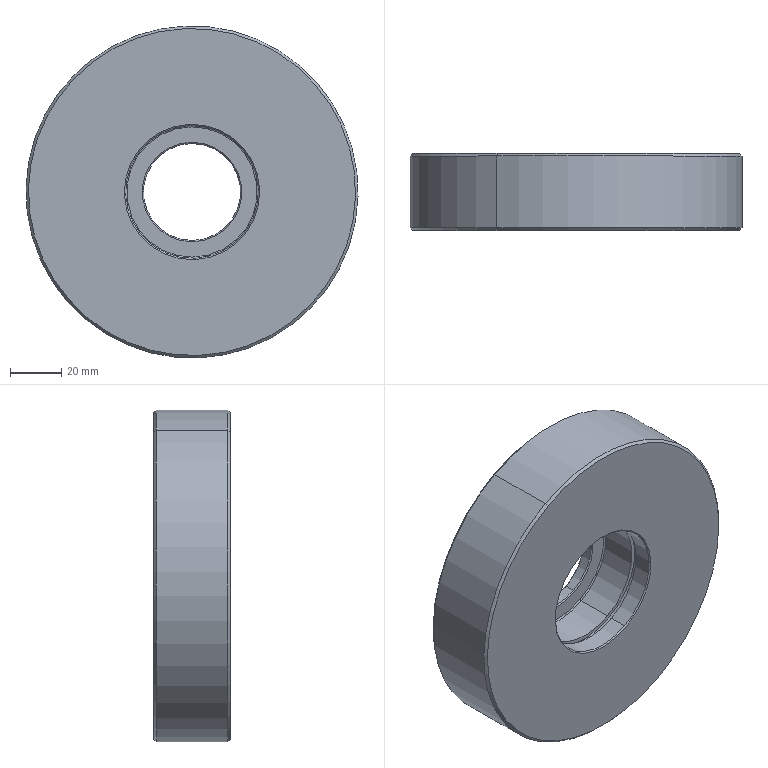Component | SolidWorks | Yk1.5.4NylonRoller-1 | 1 solid | 27 faces | box 130 x 30 x 130 mm | volume 338430 mm3 | cylinder 10 | cone 10 | plane 5 | torus 2 | commonest cylinder face diameters 52 x4 55 x2 130 x2 38 x2 | material MC Nylon
build123d program:
from build123d import *

# Parameters (mm, degrees)
SKETCH1_R           = 65
SKETCH1_R_2         = 19
BOSS_EXTRUDE1_DEPTH = 30
CHAMFER1_SIZE       = 1
SKETCH2_R           = 26
CUT_EXTRUDE2_DEPTH  = 25
CHAMFER2_SIZE       = 0.5
SKETCH3_W           = 27.5
SKETCH3_H           = 2.2
FILLET1_R           = 0.5


with BuildPart() as part:
    # Sketch1 → Boss-Extrude1 (new body)
    with BuildSketch(Plane(origin=(0, 0, 0), x_dir=(1, 0, 0), z_dir=(0, 1, 0))):
        with Locations(Location((0, 0, 0), (0, 0, 270))):
            Circle(SKETCH1_R)
        with Locations(Location((0, 0, 0), (0, 0, 270))):
            Circle(SKETCH1_R_2, mode=Mode.SUBTRACT)
    extrude(amount=BOSS_EXTRUDE1_DEPTH)

    # Chamfer1
    chamfer1_edges = [part.edges().sort_by_distance(p)[0] for p in [
        (0, 0, -65),
        (0, 30, -65),
    ]]
    chamfer(chamfer1_edges, length=CHAMFER1_SIZE)

    # Sketch2 → Cut-Extrude2 (cut)
    with BuildSketch(Plane(origin=(0, 30, 0), x_dir=(1, 0, 0), z_dir=(0, 1, 0))):
        with Locations(Location((0, 0, 0), (0, 0, 270))):
            Circle(SKETCH2_R)
    extrude(amount=-CUT_EXTRUDE2_DEPTH, mode=Mode.SUBTRACT)

    # Chamfer2
    chamfer2_edges = [part.edges().sort_by_distance(p)[0] for p in [
        (0, 5, -19),
        (0, 30, -26),
        (0, 0, -19),
    ]]
    chamfer(chamfer2_edges, length=CHAMFER2_SIZE)

    # Sketch3 → Cut-Revolve1 (revolve, cut)
    with BuildSketch(Plane.XY, mode=Mode.PRIVATE) as cut_revolve1_sk:
        with Locations((13.75, 21.1)):
            Rectangle(SKETCH3_W, SKETCH3_H)
    revolve(cut_revolve1_sk.sketch.rotate(Axis((0, 0, 0), (0, 1, 0)), 270), axis=Axis((0, 0, 0), (0, 1, 0)), mode=Mode.SUBTRACT)

    # Fillet1
    fillet1_edges = [part.edges().sort_by_distance(p)[0] for p in [
        (0, 5, -26),
    ]]
    fillet(fillet1_edges, radius=FILLET1_R)


solid = part.part

# Placed as in the assembly
solid = solid.moved(Location((98.534, -20, 23.559), (180, 0, 0)))
STEP:
#1=CARTESIAN_POINT('',(4.358,-0.9843,0.04503));
#2=VERTEX_POINT('',#1);
#3=CARTESIAN_POINT('',(3.401,-0.9843,1.81));
#4=VERTEX_POINT('',#3);
#5=CARTESIAN_POINT('',(3.879,-0.9843,0.9275));
#6=DIRECTION('',(0.,-1.,-0.));
#7=DIRECTION('',(-0.4768,0.,0.879));
#8=AXIS2_PLACEMENT_3D('',#5,#6,#7);
#9=CIRCLE('',#8,1.004);
#10=EDGE_CURVE('',#2,#4,#9,.T.);
#11=ORIENTED_EDGE('',*,*,#10,.F.);
#12=CARTESIAN_POINT('',(4.367,-1.004,0.02773));
#13=VERTEX_POINT('',#12);
#14=CARTESIAN_POINT('',(4.358,-1.004,0.04503));
#15=DIRECTION('',(-0.879,-0.,-0.4768));
#16=DIRECTION('',(-0.4768,0.,0.879));
#17=AXIS2_PLACEMENT_3D('',#14,#15,#16);
#18=CIRCLE('',#17,0.01969);
#19=EDGE_CURVE('',#2,#13,#18,.T.);
#20=ORIENTED_EDGE('',*,*,#19,.T.);
#21=CARTESIAN_POINT('',(3.391,-1.004,1.827));
#22=VERTEX_POINT('',#21);
#23=CARTESIAN_POINT('',(3.879,-1.004,0.9275));
#24=DIRECTION('',(-0.,1.,0.));
#25=DIRECTION('',(-0.4768,0.,0.879));
#26=AXIS2_PLACEMENT_3D('',#23,#24,#25);
#27=CIRCLE('',#26,1.024);
#28=EDGE_CURVE('',#22,#13,#27,.T.);
#29=ORIENTED_EDGE('',*,*,#28,.F.);
#30=CARTESIAN_POINT('',(3.401,-1.004,1.81));
#31=DIRECTION('',(0.879,0.,0.4768));
#32=DIRECTION('',(0.4768,0.,-0.879));
#33=AXIS2_PLACEMENT_3D('',#30,#31,#32);
#34=CIRCLE('',#33,0.01969);
#35=EDGE_CURVE('',#4,#22,#34,.T.);
#36=ORIENTED_EDGE('',*,*,#35,.F.);
#37=EDGE_LOOP('',(#11,#20,#29,#36));
#38=FACE_OUTER_BOUND('',#37,.T.);
#39=CARTESIAN_POINT('',(3.879,-1.004,0.9275));
#40=DIRECTION('',(0.,-1.,-0.));
#41=DIRECTION('',(-0.4768,-0.,0.879));
#42=AXIS2_PLACEMENT_3D('',#39,#40,#41);
#43=TOROIDAL_SURFACE('',#42,1.004,0.01969);
#44=ADVANCED_FACE('',(#38),#43,.F.);
#45=CARTESIAN_POINT('',(3.363,-1.661,1.879));
#46=VERTEX_POINT('',#45);
#47=CARTESIAN_POINT('',(4.395,-1.661,-0.02418));
#48=VERTEX_POINT('',#47);
#49=CARTESIAN_POINT('',(3.879,-1.661,0.9275));
#50=DIRECTION('',(-0.,1.,0.));
#51=DIRECTION('',(0.4768,0.,-0.879));
#52=AXIS2_PLACEMENT_3D('',#49,#50,#51);
#53=CIRCLE('',#52,1.083);
#54=EDGE_CURVE('',#46,#48,#53,.T.);
#55=ORIENTED_EDGE('',*,*,#54,.F.);
#56=CARTESIAN_POINT('',(3.363,-1.575,1.879));
#57=VERTEX_POINT('',#56);
#58=CARTESIAN_POINT('',(3.363,-0.7874,1.879));
#59=DIRECTION('',(-0.,1.,0.));
#60=VECTOR('',#59,39.37);
#61=LINE('',#58,#60);
#62=EDGE_CURVE('',#46,#57,#61,.T.);
#63=ORIENTED_EDGE('',*,*,#62,.T.);
#64=CARTESIAN_POINT('',(4.395,-1.575,-0.02418));
#65=VERTEX_POINT('',#64);
#66=CARTESIAN_POINT('',(3.879,-1.575,0.9275));
#67=DIRECTION('',(-0.,1.,0.));
#68=DIRECTION('',(0.4768,0.,-0.879));
#69=AXIS2_PLACEMENT_3D('',#66,#67,#68);
#70=CIRCLE('',#69,1.083);
#71=EDGE_CURVE('',#57,#65,#70,.T.);
#72=ORIENTED_EDGE('',*,*,#71,.T.);
#73=CARTESIAN_POINT('',(4.395,-0.7874,-0.02418));
#74=DIRECTION('',(-0.,1.,0.));
#75=VECTOR('',#74,39.37);
#76=LINE('',#73,#75);
#77=EDGE_CURVE('',#48,#65,#76,.T.);
#78=ORIENTED_EDGE('',*,*,#77,.F.);
#79=EDGE_LOOP('',(#55,#63,#72,#78));
#80=FACE_OUTER_BOUND('',#79,.T.);
#81=CARTESIAN_POINT('',(3.879,-0.7874,0.9275));
#82=DIRECTION('',(-0.,1.,0.));
#83=DIRECTION('',(0.4768,0.,-0.879));
#84=AXIS2_PLACEMENT_3D('',#81,#82,#83);
#85=CYLINDRICAL_SURFACE('',#84,1.083);
#86=ADVANCED_FACE('',(#80),#85,.F.);
#87=CARTESIAN_POINT('',(3.523,-0.8071,1.585));
#88=VERTEX_POINT('',#87);
#89=CARTESIAN_POINT('',(4.236,-0.8071,0.27));
#90=VERTEX_POINT('',#89);
#91=CARTESIAN_POINT('',(3.879,-0.8071,0.9275));
#92=DIRECTION('',(-0.,1.,0.));
#93=DIRECTION('',(-0.4768,0.,0.879));
#94=AXIS2_PLACEMENT_3D('',#91,#92,#93);
#95=CIRCLE('',#94,0.748);
#96=EDGE_CURVE('',#88,#90,#95,.T.);
#97=ORIENTED_EDGE('',*,*,#96,.F.);
#98=CARTESIAN_POINT('',(3.513,-0.7874,1.602));
#99=VERTEX_POINT('',#98);
#100=CARTESIAN_POINT('',(3.513,-0.7874,1.602));
#101=DIRECTION('',(-0.3371,0.7071,0.6216));
#102=VECTOR('',#101,39.37);
#103=LINE('',#100,#102);
#104=EDGE_CURVE('',#88,#99,#103,.T.);
#105=ORIENTED_EDGE('',*,*,#104,.T.);
#106=CARTESIAN_POINT('',(4.245,-0.7874,0.2527));
#107=VERTEX_POINT('',#106);
#108=CARTESIAN_POINT('',(3.879,-0.7874,0.9275));
#109=DIRECTION('',(0.,-1.,-0.));
#110=DIRECTION('',(-0.4768,0.,0.879));
#111=AXIS2_PLACEMENT_3D('',#108,#109,#110);
#112=CIRCLE('',#111,0.7677);
#113=EDGE_CURVE('',#107,#99,#112,.T.);
#114=ORIENTED_EDGE('',*,*,#113,.F.);
#115=CARTESIAN_POINT('',(4.245,-0.7874,0.2527));
#116=DIRECTION('',(0.3371,0.7071,-0.6216));
#117=VECTOR('',#116,39.37);
#118=LINE('',#115,#117);
#119=EDGE_CURVE('',#90,#107,#118,.T.);
#120=ORIENTED_EDGE('',*,*,#119,.F.);
#121=EDGE_LOOP('',(#97,#105,#114,#120));
#122=FACE_OUTER_BOUND('',#121,.T.);
#123=CARTESIAN_POINT('',(3.879,-0.7874,0.9275));
#124=DIRECTION('',(-0.,1.,0.));
#125=DIRECTION('',(0.4768,0.,-0.879));
#126=AXIS2_PLACEMENT_3D('',#123,#124,#125);
#127=CONICAL_SURFACE('',#126,0.7677,0.7854);
#128=ADVANCED_FACE('',(#122),#127,.F.);
#129=CARTESIAN_POINT('',(4.236,-0.9646,0.27));
#130=VERTEX_POINT('',#129);
#131=CARTESIAN_POINT('',(3.523,-0.9646,1.585));
#132=VERTEX_POINT('',#131);
#133=CARTESIAN_POINT('',(3.879,-0.9646,0.9275));
#134=DIRECTION('',(0.,-1.,-0.));
#135=DIRECTION('',(-0.4768,0.,0.879));
#136=AXIS2_PLACEMENT_3D('',#133,#134,#135);
#137=CIRCLE('',#136,0.748);
#138=EDGE_CURVE('',#130,#132,#137,.T.);
#139=ORIENTED_EDGE('',*,*,#138,.F.);
#140=CARTESIAN_POINT('',(4.245,-0.9843,0.2527));
#141=VERTEX_POINT('',#140);
#142=CARTESIAN_POINT('',(4.236,-0.9646,0.27));
#143=DIRECTION('',(0.3371,-0.7071,-0.6216));
#144=VECTOR('',#143,39.37);
#145=LINE('',#142,#144);
#146=EDGE_CURVE('',#130,#141,#145,.T.);
#147=ORIENTED_EDGE('',*,*,#146,.T.);
#148=CARTESIAN_POINT('',(3.513,-0.9843,1.602));
#149=VERTEX_POINT('',#148);
#150=CARTESIAN_POINT('',(3.879,-0.9843,0.9275));
#151=DIRECTION('',(-0.,1.,0.));
#152=DIRECTION('',(-0.4768,0.,0.879));
#153=AXIS2_PLACEMENT_3D('',#150,#151,#152);
#154=CIRCLE('',#153,0.7677);
#155=EDGE_CURVE('',#149,#141,#154,.T.);
#156=ORIENTED_EDGE('',*,*,#155,.F.);
#157=CARTESIAN_POINT('',(3.523,-0.9646,1.585));
#158=DIRECTION('',(-0.3371,-0.7071,0.6216));
#159=VECTOR('',#158,39.37);
#160=LINE('',#157,#159);
#161=EDGE_CURVE('',#132,#149,#160,.T.);
#162=ORIENTED_EDGE('',*,*,#161,.F.);
#163=EDGE_LOOP('',(#139,#147,#156,#162));
#164=FACE_OUTER_BOUND('',#163,.T.);
#165=CARTESIAN_POINT('',(3.879,-0.9646,0.9275));
#166=DIRECTION('',(0.,-1.,-0.));
#167=DIRECTION('',(-0.4768,0.,0.879));
#168=AXIS2_PLACEMENT_3D('',#165,#166,#167);
#169=CONICAL_SURFACE('',#168,0.748,0.7854);
#170=ADVANCED_FACE('',(#164),#169,.F.);
#171=CARTESIAN_POINT('',(4.367,-1.949,0.02773));
#172=VERTEX_POINT('',#171);
#173=CARTESIAN_POINT('',(3.391,-1.949,1.827));
#174=VERTEX_POINT('',#173);
#175=CARTESIAN_POINT('',(3.879,-1.949,0.9275));
#176=DIRECTION('',(0.,-1.,-0.));
#177=DIRECTION('',(-0.4768,0.,0.879));
#178=AXIS2_PLACEMENT_3D('',#175,#176,#177);
#179=CIRCLE('',#178,1.024);
#180=EDGE_CURVE('',#172,#174,#179,.T.);
#181=ORIENTED_EDGE('',*,*,#180,.F.);
#182=CARTESIAN_POINT('',(4.377,-1.969,0.01042));
#183=VERTEX_POINT('',#182);
#184=CARTESIAN_POINT('',(4.367,-1.949,0.02773));
#185=DIRECTION('',(0.3371,-0.7071,-0.6216));
#186=VECTOR('',#185,39.37);
#187=LINE('',#184,#186);
#188=EDGE_CURVE('',#172,#183,#187,.T.);
#189=ORIENTED_EDGE('',*,*,#188,.T.);
#190=CARTESIAN_POINT('',(3.382,-1.969,1.845));
#191=VERTEX_POINT('',#190);
#192=CARTESIAN_POINT('',(3.879,-1.969,0.9275));
#193=DIRECTION('',(-0.,1.,0.));
#194=DIRECTION('',(-0.4768,0.,0.879));
#195=AXIS2_PLACEMENT_3D('',#192,#193,#194);
#196=CIRCLE('',#195,1.043);
#197=EDGE_CURVE('',#191,#183,#196,.T.);
#198=ORIENTED_EDGE('',*,*,#197,.F.);
#199=CARTESIAN_POINT('',(3.391,-1.949,1.827));
#200=DIRECTION('',(-0.3371,-0.7071,0.6216));
#201=VECTOR('',#200,39.37);
#202=LINE('',#199,#201);
#203=EDGE_CURVE('',#174,#191,#202,.T.);
#204=ORIENTED_EDGE('',*,*,#203,.F.);
#205=EDGE_LOOP('',(#181,#189,#198,#204));
#206=FACE_OUTER_BOUND('',#205,.T.);
#207=CARTESIAN_POINT('',(3.879,-1.949,0.9275));
#208=DIRECTION('',(0.,-1.,-0.));
#209=DIRECTION('',(-0.4768,0.,0.879));
#210=AXIS2_PLACEMENT_3D('',#207,#208,#209);
#211=CONICAL_SURFACE('',#210,1.024,0.7854);
#212=ADVANCED_FACE('',(#206),#211,.F.);
#213=CARTESIAN_POINT('',(3.391,-1.661,1.827));
#214=VERTEX_POINT('',#213);
#215=CARTESIAN_POINT('',(4.367,-1.661,0.02773));
#216=VERTEX_POINT('',#215);
#217=CARTESIAN_POINT('',(3.879,-1.661,0.9275));
#218=DIRECTION('',(-0.,1.,0.));
#219=DIRECTION('',(-0.4768,0.,0.879));
#220=AXIS2_PLACEMENT_3D('',#217,#218,#219);
#221=CIRCLE('',#220,1.024);
#222=EDGE_CURVE('',#214,#216,#221,.T.);
#223=ORIENTED_EDGE('',*,*,#222,.T.);
#224=CARTESIAN_POINT('',(4.367,-0.9843,0.02773));
#225=DIRECTION('',(0.,-1.,-0.));
#226=VECTOR('',#225,39.37);
#227=LINE('',#224,#226);
#228=EDGE_CURVE('',#216,#172,#227,.T.);
#229=ORIENTED_EDGE('',*,*,#228,.T.);
#230=ORIENTED_EDGE('',*,*,#180,.T.);
#231=CARTESIAN_POINT('',(3.391,-0.9843,1.827));
#232=DIRECTION('',(0.,-1.,-0.));
#233=VECTOR('',#232,39.37);
#234=LINE('',#231,#233);
#235=EDGE_CURVE('',#214,#174,#234,.T.);
#236=ORIENTED_EDGE('',*,*,#235,.F.);
#237=EDGE_LOOP('',(#223,#229,#230,#236));
#238=FACE_OUTER_BOUND('',#237,.T.);
#239=CARTESIAN_POINT('',(3.879,-0.9843,0.9275));
#240=DIRECTION('',(0.,-1.,-0.));
#241=DIRECTION('',(-0.4768,0.,0.879));
#242=AXIS2_PLACEMENT_3D('',#239,#240,#241);
#243=CYLINDRICAL_SURFACE('',#242,1.024);
#244=ADVANCED_FACE('',(#238),#243,.F.);
#245=CARTESIAN_POINT('',(2.678,-1.969,3.142));
#246=VERTEX_POINT('',#245);
#247=CARTESIAN_POINT('',(5.081,-1.969,-1.287));
#248=VERTEX_POINT('',#247);
#249=CARTESIAN_POINT('',(3.879,-1.969,0.9275));
#250=DIRECTION('',(0.,-1.,-0.));
#251=DIRECTION('',(-0.4768,0.,0.879));
#252=AXIS2_PLACEMENT_3D('',#249,#250,#251);
#253=CIRCLE('',#252,2.52);
#254=EDGE_CURVE('',#246,#248,#253,.T.);
#255=ORIENTED_EDGE('',*,*,#254,.F.);
#256=CARTESIAN_POINT('',(2.659,-1.929,3.177));
#257=VERTEX_POINT('',#256);
#258=CARTESIAN_POINT('',(2.678,-1.969,3.142));
#259=DIRECTION('',(-0.3371,0.7071,0.6216));
#260=VECTOR('',#259,39.37);
#261=LINE('',#258,#260);
#262=EDGE_CURVE('',#246,#257,#261,.T.);
#263=ORIENTED_EDGE('',*,*,#262,.T.);
#264=CARTESIAN_POINT('',(5.099,-1.929,-1.322));
#265=VERTEX_POINT('',#264);
#266=CARTESIAN_POINT('',(3.879,-1.929,0.9275));
#267=DIRECTION('',(-0.,1.,0.));
#268=DIRECTION('',(-0.4768,0.,0.879));
#269=AXIS2_PLACEMENT_3D('',#266,#267,#268);
#270=CIRCLE('',#269,2.559);
#271=EDGE_CURVE('',#265,#257,#270,.T.);
#272=ORIENTED_EDGE('',*,*,#271,.F.);
#273=CARTESIAN_POINT('',(5.081,-1.969,-1.287));
#274=DIRECTION('',(0.3371,0.7071,-0.6216));
#275=VECTOR('',#274,39.37);
#276=LINE('',#273,#275);
#277=EDGE_CURVE('',#248,#265,#276,.T.);
#278=ORIENTED_EDGE('',*,*,#277,.F.);
#279=EDGE_LOOP('',(#255,#263,#272,#278));
#280=FACE_OUTER_BOUND('',#279,.T.);
#281=CARTESIAN_POINT('',(3.879,-1.969,0.9275));
#282=DIRECTION('',(-0.,1.,0.));
#283=DIRECTION('',(0.4768,0.,-0.879));
#284=AXIS2_PLACEMENT_3D('',#281,#282,#283);
#285=CONICAL_SURFACE('',#284,2.52,0.7854);
#286=ADVANCED_FACE('',(#280),#285,.T.);
#287=CARTESIAN_POINT('',(5.081,-0.7874,-1.287));
#288=VERTEX_POINT('',#287);
#289=CARTESIAN_POINT('',(2.678,-0.7874,3.142));
#290=VERTEX_POINT('',#289);
#291=CARTESIAN_POINT('',(3.879,-0.7874,0.9275));
#292=DIRECTION('',(-0.,1.,0.));
#293=DIRECTION('',(-0.4768,0.,0.879));
#294=AXIS2_PLACEMENT_3D('',#291,#292,#293);
#295=CIRCLE('',#294,2.52);
#296=EDGE_CURVE('',#288,#290,#295,.T.);
#297=ORIENTED_EDGE('',*,*,#296,.F.);
#298=CARTESIAN_POINT('',(5.099,-0.8268,-1.322));
#299=VERTEX_POINT('',#298);
#300=CARTESIAN_POINT('',(5.099,-0.8268,-1.322));
#301=DIRECTION('',(0.3371,-0.7071,-0.6216));
#302=VECTOR('',#301,39.37);
#303=LINE('',#300,#302);
#304=EDGE_CURVE('',#288,#299,#303,.T.);
#305=ORIENTED_EDGE('',*,*,#304,.T.);
#306=CARTESIAN_POINT('',(2.659,-0.8268,3.177));
#307=VERTEX_POINT('',#306);
#308=CARTESIAN_POINT('',(3.879,-0.8268,0.9275));
#309=DIRECTION('',(0.,-1.,-0.));
#310=DIRECTION('',(-0.4768,0.,0.879));
#311=AXIS2_PLACEMENT_3D('',#308,#309,#310);
#312=CIRCLE('',#311,2.559);
#313=EDGE_CURVE('',#307,#299,#312,.T.);
#314=ORIENTED_EDGE('',*,*,#313,.F.);
#315=CARTESIAN_POINT('',(2.659,-0.8268,3.177));
#316=DIRECTION('',(-0.3371,-0.7071,0.6216));
#317=VECTOR('',#316,39.37);
#318=LINE('',#315,#317);
#319=EDGE_CURVE('',#290,#307,#318,.T.);
#320=ORIENTED_EDGE('',*,*,#319,.F.);
#321=EDGE_LOOP('',(#297,#305,#314,#320));
#322=FACE_OUTER_BOUND('',#321,.T.);
#323=CARTESIAN_POINT('',(3.879,-0.8268,0.9275));
#324=DIRECTION('',(0.,-1.,-0.));
#325=DIRECTION('',(-0.4768,0.,0.879));
#326=AXIS2_PLACEMENT_3D('',#323,#324,#325);
#327=CONICAL_SURFACE('',#326,2.559,0.7854);
#328=ADVANCED_FACE('',(#322),#327,.T.);
#329=ORIENTED_EDGE('',*,*,#271,.T.);
#330=CARTESIAN_POINT('',(2.659,-1.969,3.177));
#331=DIRECTION('',(-0.,1.,0.));
#332=VECTOR('',#331,39.37);
#333=LINE('',#330,#332);
#334=EDGE_CURVE('',#257,#307,#333,.T.);
#335=ORIENTED_EDGE('',*,*,#334,.T.);
#336=ORIENTED_EDGE('',*,*,#313,.T.);
#337=CARTESIAN_POINT('',(5.099,-1.969,-1.322));
#338=DIRECTION('',(-0.,1.,0.));
#339=VECTOR('',#338,39.37);
#340=LINE('',#337,#339);
#341=EDGE_CURVE('',#265,#299,#340,.T.);
#342=ORIENTED_EDGE('',*,*,#341,.F.);
#343=EDGE_LOOP('',(#329,#335,#336,#342));
#344=FACE_OUTER_BOUND('',#343,.T.);
#345=CARTESIAN_POINT('',(3.879,-1.969,0.9275));
#346=DIRECTION('',(-0.,1.,0.));
#347=DIRECTION('',(0.4768,0.,-0.879));
#348=AXIS2_PLACEMENT_3D('',#345,#346,#347);
#349=CYLINDRICAL_SURFACE('',#348,2.559);
#350=ADVANCED_FACE('',(#344),#349,.T.);
#351=ORIENTED_EDGE('',*,*,#138,.T.);
#352=CARTESIAN_POINT('',(3.523,-1.969,1.585));
#353=DIRECTION('',(-0.,1.,0.));
#354=VECTOR('',#353,39.37);
#355=LINE('',#352,#354);
#356=EDGE_CURVE('',#132,#88,#355,.T.);
#357=ORIENTED_EDGE('',*,*,#356,.T.);
#358=ORIENTED_EDGE('',*,*,#96,.T.);
#359=CARTESIAN_POINT('',(4.236,-1.969,0.27));
#360=DIRECTION('',(-0.,1.,0.));
#361=VECTOR('',#360,39.37);
#362=LINE('',#359,#361);
#363=EDGE_CURVE('',#130,#90,#362,.T.);
#364=ORIENTED_EDGE('',*,*,#363,.F.);
#365=EDGE_LOOP('',(#351,#357,#358,#364));
#366=FACE_OUTER_BOUND('',#365,.T.);
#367=CARTESIAN_POINT('',(3.879,-1.969,0.9275));
#368=DIRECTION('',(-0.,1.,0.));
#369=DIRECTION('',(0.4768,0.,-0.879));
#370=AXIS2_PLACEMENT_3D('',#367,#368,#369);
#371=CYLINDRICAL_SURFACE('',#370,0.748);
#372=ADVANCED_FACE('',(#366),#371,.F.);
#373=ORIENTED_EDGE('',*,*,#28,.T.);
#374=CARTESIAN_POINT('',(4.367,-1.575,0.02773));
#375=VERTEX_POINT('',#374);
#376=CARTESIAN_POINT('',(4.367,-0.9843,0.02773));
#377=DIRECTION('',(0.,-1.,-0.));
#378=VECTOR('',#377,39.37);
#379=LINE('',#376,#378);
#380=EDGE_CURVE('',#13,#375,#379,.T.);
#381=ORIENTED_EDGE('',*,*,#380,.T.);
#382=CARTESIAN_POINT('',(3.391,-1.575,1.827));
#383=VERTEX_POINT('',#382);
#384=CARTESIAN_POINT('',(3.879,-1.575,0.9275));
#385=DIRECTION('',(0.,-1.,-0.));
#386=DIRECTION('',(0.4768,0.,-0.879));
#387=AXIS2_PLACEMENT_3D('',#384,#385,#386);
#388=CIRCLE('',#387,1.024);
#389=EDGE_CURVE('',#375,#383,#388,.T.);
#390=ORIENTED_EDGE('',*,*,#389,.T.);
#391=CARTESIAN_POINT('',(3.391,-0.9843,1.827));
#392=DIRECTION('',(0.,-1.,-0.));
#393=VECTOR('',#392,39.37);
#394=LINE('',#391,#393);
#395=EDGE_CURVE('',#22,#383,#394,.T.);
#396=ORIENTED_EDGE('',*,*,#395,.F.);
#397=EDGE_LOOP('',(#373,#381,#390,#396));
#398=FACE_OUTER_BOUND('',#397,.T.);
#399=CARTESIAN_POINT('',(3.879,-0.9843,0.9275));
#400=DIRECTION('',(0.,-1.,-0.));
#401=DIRECTION('',(-0.4768,0.,0.879));
#402=AXIS2_PLACEMENT_3D('',#399,#400,#401);
#403=CYLINDRICAL_SURFACE('',#402,1.024);
#404=ADVANCED_FACE('',(#398),#403,.F.);
#405=ORIENTED_EDGE('',*,*,#380,.F.);
#406=CARTESIAN_POINT('',(3.879,-1.004,0.9275));
#407=DIRECTION('',(-0.,1.,0.));
#408=DIRECTION('',(-0.4768,0.,0.879));
#409=AXIS2_PLACEMENT_3D('',#406,#407,#408);
#410=CIRCLE('',#409,1.024);
#411=EDGE_CURVE('',#13,#22,#410,.T.);
#412=ORIENTED_EDGE('',*,*,#411,.T.);
#413=ORIENTED_EDGE('',*,*,#395,.T.);
#414=CARTESIAN_POINT('',(3.879,-1.575,0.9275));
#415=DIRECTION('',(0.,-1.,-0.));
#416=DIRECTION('',(0.4768,0.,-0.879));
#417=AXIS2_PLACEMENT_3D('',#414,#415,#416);
#418=CIRCLE('',#417,1.024);
#419=EDGE_CURVE('',#383,#375,#418,.T.);
#420=ORIENTED_EDGE('',*,*,#419,.T.);
#421=EDGE_LOOP('',(#405,#412,#413,#420));
#422=FACE_OUTER_BOUND('',#421,.T.);
#423=CARTESIAN_POINT('',(3.879,-0.9843,0.9275));
#424=DIRECTION('',(0.,-1.,-0.));
#425=DIRECTION('',(-0.4768,0.,0.879));
#426=AXIS2_PLACEMENT_3D('',#423,#424,#425);
#427=CYLINDRICAL_SURFACE('',#426,1.024);
#428=ADVANCED_FACE('',(#422),#427,.F.);
#429=ORIENTED_EDGE('',*,*,#356,.F.);
#430=CARTESIAN_POINT('',(3.879,-0.9646,0.9275));
#431=DIRECTION('',(0.,-1.,-0.));
#432=DIRECTION('',(-0.4768,0.,0.879));
#433=AXIS2_PLACEMENT_3D('',#430,#431,#432);
#434=CIRCLE('',#433,0.748);
#435=EDGE_CURVE('',#132,#130,#434,.T.);
#436=ORIENTED_EDGE('',*,*,#435,.T.);
#437=ORIENTED_EDGE('',*,*,#363,.T.);
#438=CARTESIAN_POINT('',(3.879,-0.8071,0.9275));
#439=DIRECTION('',(-0.,1.,0.));
#440=DIRECTION('',(-0.4768,0.,0.879));
#441=AXIS2_PLACEMENT_3D('',#438,#439,#440);
#442=CIRCLE('',#441,0.748);
#443=EDGE_CURVE('',#90,#88,#442,.T.);
#444=ORIENTED_EDGE('',*,*,#443,.T.);
#445=EDGE_LOOP('',(#429,#436,#437,#444));
#446=FACE_OUTER_BOUND('',#445,.T.);
#447=CARTESIAN_POINT('',(3.879,-1.969,0.9275));
#448=DIRECTION('',(-0.,1.,0.));
#449=DIRECTION('',(0.4768,0.,-0.879));
#450=AXIS2_PLACEMENT_3D('',#447,#448,#449);
#451=CYLINDRICAL_SURFACE('',#450,0.748);
#452=ADVANCED_FACE('',(#446),#451,.F.);
#453=ORIENTED_EDGE('',*,*,#197,.T.);
#454=CARTESIAN_POINT('',(3.879,-1.969,0.9275));
#455=DIRECTION('',(-0.,1.,0.));
#456=DIRECTION('',(-0.4768,0.,0.879));
#457=AXIS2_PLACEMENT_3D('',#454,#455,#456);
#458=CIRCLE('',#457,1.043);
#459=EDGE_CURVE('',#183,#191,#458,.T.);
#460=ORIENTED_EDGE('',*,*,#459,.T.);
#461=EDGE_LOOP('',(#453,#460));
#462=FACE_BOUND('',#461,.T.);
#463=CARTESIAN_POINT('',(3.879,-1.969,0.9275));
#464=DIRECTION('',(0.,-1.,-0.));
#465=DIRECTION('',(-0.4768,0.,0.879));
#466=AXIS2_PLACEMENT_3D('',#463,#464,#465);
#467=CIRCLE('',#466,2.52);
#468=EDGE_CURVE('',#248,#246,#467,.T.);
#469=ORIENTED_EDGE('',*,*,#468,.T.);
#470=ORIENTED_EDGE('',*,*,#254,.T.);
#471=EDGE_LOOP('',(#469,#470));
#472=FACE_OUTER_BOUND('',#471,.T.);
#473=CARTESIAN_POINT('',(3.879,-1.969,0.9275));
#474=DIRECTION('',(0.,-1.,-0.));
#475=DIRECTION('',(-0.4768,-0.,0.879));
#476=AXIS2_PLACEMENT_3D('',#473,#474,#475);
#477=PLANE('',#476);
#478=ADVANCED_FACE('',(#462,#472),#477,.T.);
#479=ORIENTED_EDGE('',*,*,#113,.T.);
#480=CARTESIAN_POINT('',(3.879,-0.7874,0.9275));
#481=DIRECTION('',(0.,-1.,-0.));
#482=DIRECTION('',(-0.4768,0.,0.879));
#483=AXIS2_PLACEMENT_3D('',#480,#481,#482);
#484=CIRCLE('',#483,0.7677);
#485=EDGE_CURVE('',#99,#107,#484,.T.);
#486=ORIENTED_EDGE('',*,*,#485,.T.);
#487=EDGE_LOOP('',(#479,#486));
#488=FACE_BOUND('',#487,.T.);
#489=CARTESIAN_POINT('',(3.879,-0.7874,0.9275));
#490=DIRECTION('',(-0.,1.,0.));
#491=DIRECTION('',(-0.4768,0.,0.879));
#492=AXIS2_PLACEMENT_3D('',#489,#490,#491);
#493=CIRCLE('',#492,2.52);
#494=EDGE_CURVE('',#290,#288,#493,.T.);
#495=ORIENTED_EDGE('',*,*,#494,.T.);
#496=ORIENTED_EDGE('',*,*,#296,.T.);
#497=EDGE_LOOP('',(#495,#496));
#498=FACE_OUTER_BOUND('',#497,.T.);
#499=CARTESIAN_POINT('',(3.879,-0.7874,0.9275));
#500=DIRECTION('',(0.,-1.,-0.));
#501=DIRECTION('',(-0.4768,-0.,0.879));
#502=AXIS2_PLACEMENT_3D('',#499,#500,#501);
#503=PLANE('',#502);
#504=ADVANCED_FACE('',(#488,#498),#503,.F.);
#505=ORIENTED_EDGE('',*,*,#334,.F.);
#506=CARTESIAN_POINT('',(3.879,-1.929,0.9275));
#507=DIRECTION('',(-0.,1.,0.));
#508=DIRECTION('',(-0.4768,0.,0.879));
#509=AXIS2_PLACEMENT_3D('',#506,#507,#508);
#510=CIRCLE('',#509,2.559);
#511=EDGE_CURVE('',#257,#265,#510,.T.);
#512=ORIENTED_EDGE('',*,*,#511,.T.);
#513=ORIENTED_EDGE('',*,*,#341,.T.);
#514=CARTESIAN_POINT('',(3.879,-0.8268,0.9275));
#515=DIRECTION('',(0.,-1.,-0.));
#516=DIRECTION('',(-0.4768,0.,0.879));
#517=AXIS2_PLACEMENT_3D('',#514,#515,#516);
#518=CIRCLE('',#517,2.559);
#519=EDGE_CURVE('',#299,#307,#518,.T.);
#520=ORIENTED_EDGE('',*,*,#519,.T.);
#521=EDGE_LOOP('',(#505,#512,#513,#520));
#522=FACE_OUTER_BOUND('',#521,.T.);
#523=CARTESIAN_POINT('',(3.879,-1.969,0.9275));
#524=DIRECTION('',(-0.,1.,0.));
#525=DIRECTION('',(0.4768,0.,-0.879));
#526=AXIS2_PLACEMENT_3D('',#523,#524,#525);
#527=CYLINDRICAL_SURFACE('',#526,2.559);
#528=ADVANCED_FACE('',(#522),#527,.T.);
#529=ORIENTED_EDGE('',*,*,#304,.F.);
#530=ORIENTED_EDGE('',*,*,#494,.F.);
#531=ORIENTED_EDGE('',*,*,#319,.T.);
#532=ORIENTED_EDGE('',*,*,#519,.F.);
#533=EDGE_LOOP('',(#529,#530,#531,#532));
#534=FACE_OUTER_BOUND('',#533,.T.);
#535=CARTESIAN_POINT('',(3.879,-0.8268,0.9275));
#536=DIRECTION('',(0.,-1.,-0.));
#537=DIRECTION('',(-0.4768,0.,0.879));
#538=AXIS2_PLACEMENT_3D('',#535,#536,#537);
#539=CONICAL_SURFACE('',#538,2.559,0.7854);
#540=ADVANCED_FACE('',(#534),#539,.T.);
#541=ORIENTED_EDGE('',*,*,#262,.F.);
#542=ORIENTED_EDGE('',*,*,#468,.F.);
#543=ORIENTED_EDGE('',*,*,#277,.T.);
#544=ORIENTED_EDGE('',*,*,#511,.F.);
#545=EDGE_LOOP('',(#541,#542,#543,#544));
#546=FACE_OUTER_BOUND('',#545,.T.);
#547=CARTESIAN_POINT('',(3.879,-1.969,0.9275));
#548=DIRECTION('',(-0.,1.,0.));
#549=DIRECTION('',(0.4768,0.,-0.879));
#550=AXIS2_PLACEMENT_3D('',#547,#548,#549);
#551=CONICAL_SURFACE('',#550,2.52,0.7854);
#552=ADVANCED_FACE('',(#546),#551,.T.);
#553=ORIENTED_EDGE('',*,*,#228,.F.);
#554=CARTESIAN_POINT('',(3.879,-1.661,0.9275));
#555=DIRECTION('',(-0.,1.,0.));
#556=DIRECTION('',(-0.4768,0.,0.879));
#557=AXIS2_PLACEMENT_3D('',#554,#555,#556);
#558=CIRCLE('',#557,1.024);
#559=EDGE_CURVE('',#216,#214,#558,.T.);
#560=ORIENTED_EDGE('',*,*,#559,.T.);
#561=ORIENTED_EDGE('',*,*,#235,.T.);
#562=CARTESIAN_POINT('',(3.879,-1.949,0.9275));
#563=DIRECTION('',(0.,-1.,-0.));
#564=DIRECTION('',(-0.4768,0.,0.879));
#565=AXIS2_PLACEMENT_3D('',#562,#563,#564);
#566=CIRCLE('',#565,1.024);
#567=EDGE_CURVE('',#174,#172,#566,.T.);
#568=ORIENTED_EDGE('',*,*,#567,.T.);
#569=EDGE_LOOP('',(#553,#560,#561,#568));
#570=FACE_OUTER_BOUND('',#569,.T.);
#571=CARTESIAN_POINT('',(3.879,-0.9843,0.9275));
#572=DIRECTION('',(0.,-1.,-0.));
#573=DIRECTION('',(-0.4768,0.,0.879));
#574=AXIS2_PLACEMENT_3D('',#571,#572,#573);
#575=CYLINDRICAL_SURFACE('',#574,1.024);
#576=ADVANCED_FACE('',(#570),#575,.F.);
#577=CARTESIAN_POINT('',(3.879,-0.9843,0.9275));
#578=DIRECTION('',(0.,-1.,-0.));
#579=DIRECTION('',(-0.4768,0.,0.879));
#580=AXIS2_PLACEMENT_3D('',#577,#578,#579);
#581=CIRCLE('',#580,1.004);
#582=EDGE_CURVE('',#4,#2,#581,.T.);
#583=ORIENTED_EDGE('',*,*,#582,.T.);
#584=ORIENTED_EDGE('',*,*,#10,.T.);
#585=EDGE_LOOP('',(#583,#584));
#586=FACE_OUTER_BOUND('',#585,.T.);
#587=ORIENTED_EDGE('',*,*,#155,.T.);
#588=CARTESIAN_POINT('',(3.879,-0.9843,0.9275));
#589=DIRECTION('',(-0.,1.,0.));
#590=DIRECTION('',(-0.4768,0.,0.879));
#591=AXIS2_PLACEMENT_3D('',#588,#589,#590);
#592=CIRCLE('',#591,0.7677);
#593=EDGE_CURVE('',#141,#149,#592,.T.);
#594=ORIENTED_EDGE('',*,*,#593,.T.);
#595=EDGE_LOOP('',(#587,#594));
#596=FACE_BOUND('',#595,.T.);
#597=CARTESIAN_POINT('',(3.879,-0.9843,0.9275));
#598=DIRECTION('',(0.,-1.,-0.));
#599=DIRECTION('',(-0.4768,-0.,0.879));
#600=AXIS2_PLACEMENT_3D('',#597,#598,#599);
#601=PLANE('',#600);
#602=ADVANCED_FACE('',(#586,#596),#601,.T.);
#603=ORIENTED_EDGE('',*,*,#188,.F.);
#604=ORIENTED_EDGE('',*,*,#567,.F.);
#605=ORIENTED_EDGE('',*,*,#203,.T.);
#606=ORIENTED_EDGE('',*,*,#459,.F.);
#607=EDGE_LOOP('',(#603,#604,#605,#606));
#608=FACE_OUTER_BOUND('',#607,.T.);
#609=CARTESIAN_POINT('',(3.879,-1.949,0.9275));
#610=DIRECTION('',(0.,-1.,-0.));
#611=DIRECTION('',(-0.4768,0.,0.879));
#612=AXIS2_PLACEMENT_3D('',#609,#610,#611);
#613=CONICAL_SURFACE('',#612,1.024,0.7854);
#614=ADVANCED_FACE('',(#608),#613,.F.);
#615=ORIENTED_EDGE('',*,*,#146,.F.);
#616=ORIENTED_EDGE('',*,*,#435,.F.);
#617=ORIENTED_EDGE('',*,*,#161,.T.);
#618=ORIENTED_EDGE('',*,*,#593,.F.);
#619=EDGE_LOOP('',(#615,#616,#617,#618));
#620=FACE_OUTER_BOUND('',#619,.T.);
#621=CARTESIAN_POINT('',(3.879,-0.9646,0.9275));
#622=DIRECTION('',(0.,-1.,-0.));
#623=DIRECTION('',(-0.4768,0.,0.879));
#624=AXIS2_PLACEMENT_3D('',#621,#622,#623);
#625=CONICAL_SURFACE('',#624,0.748,0.7854);
#626=ADVANCED_FACE('',(#620),#625,.F.);
#627=ORIENTED_EDGE('',*,*,#104,.F.);
#628=ORIENTED_EDGE('',*,*,#443,.F.);
#629=ORIENTED_EDGE('',*,*,#119,.T.);
#630=ORIENTED_EDGE('',*,*,#485,.F.);
#631=EDGE_LOOP('',(#627,#628,#629,#630));
#632=FACE_OUTER_BOUND('',#631,.T.);
#633=CARTESIAN_POINT('',(3.879,-0.7874,0.9275));
#634=DIRECTION('',(-0.,1.,0.));
#635=DIRECTION('',(0.4768,0.,-0.879));
#636=AXIS2_PLACEMENT_3D('',#633,#634,#635);
#637=CONICAL_SURFACE('',#636,0.7677,0.7854);
#638=ADVANCED_FACE('',(#632),#637,.F.);
#639=CARTESIAN_POINT('',(3.879,-1.575,0.9275));
#640=DIRECTION('',(-0.,1.,0.));
#641=DIRECTION('',(0.4768,0.,-0.879));
#642=AXIS2_PLACEMENT_3D('',#639,#640,#641);
#643=CIRCLE('',#642,1.083);
#644=EDGE_CURVE('',#65,#57,#643,.T.);
#645=ORIENTED_EDGE('',*,*,#644,.F.);
#646=ORIENTED_EDGE('',*,*,#71,.F.);
#647=EDGE_LOOP('',(#645,#646));
#648=FACE_OUTER_BOUND('',#647,.T.);
#649=ORIENTED_EDGE('',*,*,#419,.F.);
#650=ORIENTED_EDGE('',*,*,#389,.F.);
#651=EDGE_LOOP('',(#649,#650));
#652=FACE_BOUND('',#651,.T.);
#653=CARTESIAN_POINT('',(3.879,-1.575,0.9275));
#654=DIRECTION('',(-0.,1.,0.));
#655=DIRECTION('',(0.4768,0.,-0.879));
#656=AXIS2_PLACEMENT_3D('',#653,#654,#655);
#657=PLANE('',#656);
#658=ADVANCED_FACE('',(#648,#652),#657,.F.);
#659=CARTESIAN_POINT('',(3.879,-1.661,0.9275));
#660=DIRECTION('',(-0.,1.,0.));
#661=DIRECTION('',(0.4768,0.,-0.879));
#662=AXIS2_PLACEMENT_3D('',#659,#660,#661);
#663=CIRCLE('',#662,1.083);
#664=EDGE_CURVE('',#48,#46,#663,.T.);
#665=ORIENTED_EDGE('',*,*,#664,.T.);
#666=ORIENTED_EDGE('',*,*,#54,.T.);
#667=EDGE_LOOP('',(#665,#666));
#668=FACE_OUTER_BOUND('',#667,.T.);
#669=ORIENTED_EDGE('',*,*,#222,.F.);
#670=ORIENTED_EDGE('',*,*,#559,.F.);
#671=EDGE_LOOP('',(#669,#670));
#672=FACE_BOUND('',#671,.T.);
#673=CARTESIAN_POINT('',(2.928,-1.661,0.4113));
#674=DIRECTION('',(0.,-1.,-0.));
#675=DIRECTION('',(-0.4768,-0.,0.879));
#676=AXIS2_PLACEMENT_3D('',#673,#674,#675);
#677=PLANE('',#676);
#678=ADVANCED_FACE('',(#668,#672),#677,.F.);
#679=ORIENTED_EDGE('',*,*,#62,.F.);
#680=ORIENTED_EDGE('',*,*,#664,.F.);
#681=ORIENTED_EDGE('',*,*,#77,.T.);
#682=ORIENTED_EDGE('',*,*,#644,.T.);
#683=EDGE_LOOP('',(#679,#680,#681,#682));
#684=FACE_OUTER_BOUND('',#683,.T.);
#685=CARTESIAN_POINT('',(3.879,-0.7874,0.9275));
#686=DIRECTION('',(-0.,1.,0.));
#687=DIRECTION('',(0.4768,0.,-0.879));
#688=AXIS2_PLACEMENT_3D('',#685,#686,#687);
#689=CYLINDRICAL_SURFACE('',#688,1.083);
#690=ADVANCED_FACE('',(#684),#689,.F.);
#691=ORIENTED_EDGE('',*,*,#19,.F.);
#692=ORIENTED_EDGE('',*,*,#582,.F.);
#693=ORIENTED_EDGE('',*,*,#35,.T.);
#694=ORIENTED_EDGE('',*,*,#411,.F.);
#695=EDGE_LOOP('',(#691,#692,#693,#694));
#696=FACE_OUTER_BOUND('',#695,.T.);
#697=CARTESIAN_POINT('',(3.879,-1.004,0.9275));
#698=DIRECTION('',(0.,-1.,-0.));
#699=DIRECTION('',(-0.4768,-0.,0.879));
#700=AXIS2_PLACEMENT_3D('',#697,#698,#699);
#701=TOROIDAL_SURFACE('',#700,1.004,0.01969);
#702=ADVANCED_FACE('',(#696),#701,.F.);
#703=CLOSED_SHELL('',(#44,#86,#128,#170,#212,#244,#286,#328,#350,#372,#404,#428,#452,#478,#504,#528,#540,#552,#576,#602,#614,#626,#638,#658,#678,#690,#702));
#704=MANIFOLD_SOLID_BREP('',#703);
#705=CARTESIAN_POINT('',(0.,0.,0.));
#706=DIRECTION('',(0.,0.,1.));
#707=DIRECTION('',(1.,0.,0.));
#708=AXIS2_PLACEMENT_3D('',#705,#706,#707);
#709=(LENGTH_UNIT()NAMED_UNIT(*)SI_UNIT($,.METRE.));
#710=LENGTH_MEASURE_WITH_UNIT(LENGTH_MEASURE(0.0254),#709);
#711=DIMENSIONAL_EXPONENTS(1.,0.,0.,0.,0.,0.,0.);
#712=(CONVERSION_BASED_UNIT('',#710)LENGTH_UNIT()NAMED_UNIT(#711));
#713=UNCERTAINTY_MEASURE_WITH_UNIT(LENGTH_MEASURE(0.00001),#712,'','');
#714=(NAMED_UNIT(*)PLANE_ANGLE_UNIT()SI_UNIT($,.RADIAN.));
#715=(NAMED_UNIT(*)SI_UNIT($,.STERADIAN.)SOLID_ANGLE_UNIT());
#716=(GEOMETRIC_REPRESENTATION_CONTEXT(3)GLOBAL_UNCERTAINTY_ASSIGNED_CONTEXT((#713))GLOBAL_UNIT_ASSIGNED_CONTEXT((#712,#714,#715))REPRESENTATION_CONTEXT('',''));
#717=ADVANCED_BREP_SHAPE_REPRESENTATION('',(#704,#708),#716);
#718=COLOUR_RGB('',0.7922,0.8196,0.9333);
#719=FILL_AREA_STYLE_COLOUR('',#718);
#720=FILL_AREA_STYLE('',(#719));
#721=SURFACE_STYLE_FILL_AREA(#720);
#722=SURFACE_SIDE_STYLE('',(#721));
#723=SURFACE_STYLE_USAGE(.BOTH.,#722);
#724=PRESENTATION_STYLE_ASSIGNMENT((#723));
#725=STYLED_ITEM('',(#724),#704);
#726=(LENGTH_UNIT()NAMED_UNIT(*)SI_UNIT($,.METRE.));
#727=LENGTH_MEASURE_WITH_UNIT(LENGTH_MEASURE(0.0254),#726);
#728=DIMENSIONAL_EXPONENTS(1.,0.,0.,0.,0.,0.,0.);
#729=(CONVERSION_BASED_UNIT('',#727)LENGTH_UNIT()NAMED_UNIT(#728));
#730=UNCERTAINTY_MEASURE_WITH_UNIT(LENGTH_MEASURE(0.00001),#729,'','');
#731=(NAMED_UNIT(*)PLANE_ANGLE_UNIT()SI_UNIT($,.RADIAN.));
#732=(NAMED_UNIT(*)SI_UNIT($,.STERADIAN.)SOLID_ANGLE_UNIT());
#733=(GEOMETRIC_REPRESENTATION_CONTEXT(3)GLOBAL_UNCERTAINTY_ASSIGNED_CONTEXT((#730))GLOBAL_UNIT_ASSIGNED_CONTEXT((#729,#731,#732))REPRESENTATION_CONTEXT('',''));
#734=MECHANICAL_DESIGN_GEOMETRIC_PRESENTATION_REPRESENTATION('',(#725),#733);
#735=PRESENTATION_LAYER_ASSIGNMENT('','',(#725));